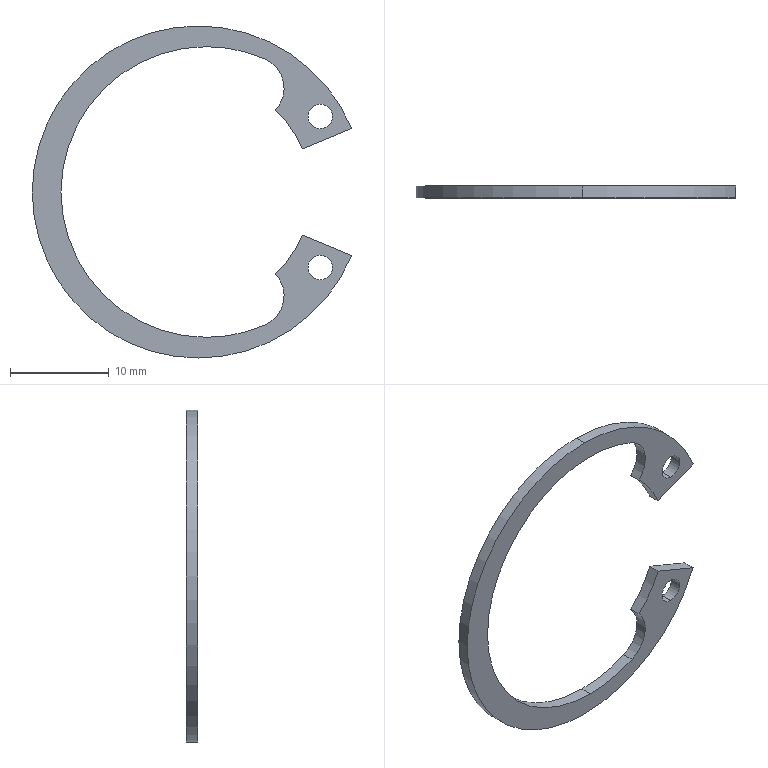Component | SolidWorks | 8TC-A15004-83-00-16_circlips for hole--type b gb-1 | 1 solid | 18 faces | volume 282 mm3 | cylinder 14 | plane 4 | commonest cylinder face diameters 2.5 x4 29.5 x3 33.7 x3 22.82 x2 6.4 x2